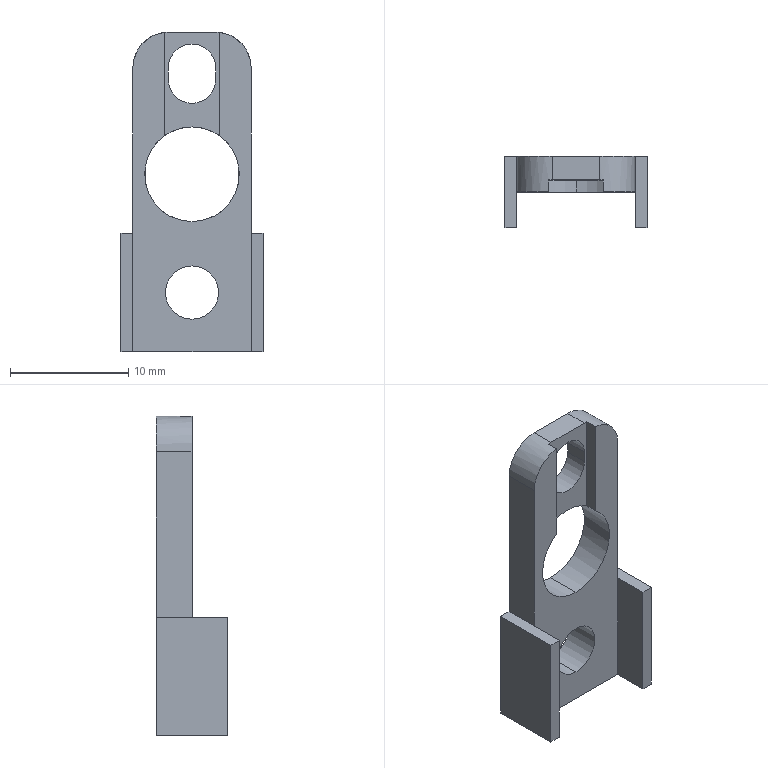Component | SolidWorks | BearingHousingAssembly-1_JawBuckleJaw-1 | 1 solid | 28 faces | box 12 x 6 x 27 mm | volume 649 mm3 | plane 19 | cylinder 9 | commonest cylinder face diameters 4 x3 8 x2 4.5 x2 6 x2
build123d program:
from build123d import *

# Parameters (mm, degrees)
SKETCH1_W                  = 27
SKETCH1_H                  = 10
BOSS_EXTRUDE1_DEPTH        = 3
F_4_5_4_5_DIAMETER_HOLE1_D = 4.5
SKETCH4_W                  = 6
SKETCH4_H                  = 1
BOSS_EXTRUDE2_DEPTH        = 10
SKETCH5_R                  = 4
CUT_EXTRUDE1_DEPTH         = 29.302
FILLET1_R                  = 3
CUT_EXTRUDE2_DEPTH         = 29.302
SKETCH7_W                  = 10.742
SKETCH7_H                  = 4.6
CUT_EXTRUDE3_DEPTH         = 1


with BuildPart() as part:
    # Sketch1 → Boss-Extrude1 (new body)
    with BuildSketch(Plane.XY):
        with Locations((13.5, 0)):
            Rectangle(SKETCH1_W, SKETCH1_H)
    extrude(amount=BOSS_EXTRUDE1_DEPTH)

    # 4.5 _4.5_ Diameter Hole1 (through all)
    with Locations(Plane(origin=(0, 0, 0), x_dir=(-1, 0, 0), z_dir=(0, 0, -1))):
        with Locations((-5, 0)):
            Hole(F_4_5_4_5_DIAMETER_HOLE1_D / 2)

    # Sketch4 → Boss-Extrude2 (add)
    with BuildSketch(Plane.ZY):
        with Locations((0, 5.5)):
            Rectangle(SKETCH4_W, SKETCH4_H)
        with Locations((0, -5.5)):
            Rectangle(SKETCH4_W, SKETCH4_H)
    extrude(amount=-BOSS_EXTRUDE2_DEPTH)

    # Sketch5 → Cut-Extrude1 (cut, through all)
    with BuildSketch(Plane.XY.offset(3)):
        with Locations((15, 0)):
            Circle(SKETCH5_R)
    extrude(amount=-CUT_EXTRUDE1_DEPTH, mode=Mode.SUBTRACT)

    # Fillet1
    fillet1_edges = [part.edges().sort_by_distance(p)[0] for p in [
        (27, -5, 1.5),
        (27, 5, 1.5),
    ]]
    fillet(fillet1_edges, radius=FILLET1_R)

    # Sketch6 → Cut-Extrude2 (cut, through all)
    with BuildSketch(Plane.XY.offset(3)):
        with BuildLine():
            Line((23, 2), (24, 2))
            ThreePointArc((24, 2), (26, 0), (24, -2))
            Line((24, -2), (23, -2))
            ThreePointArc((23, -2), (21, 0), (23, 2))
        make_face()
    extrude(amount=-CUT_EXTRUDE2_DEPTH, mode=Mode.SUBTRACT)

    # Sketch7 → Cut-Extrude3 (cut)
    with BuildSketch(Plane(origin=(0, 0, 0), x_dir=(-1, 0, 0), z_dir=(0, 0, -1))):
        with Locations((-23.371, 0)):
            Rectangle(SKETCH7_W, SKETCH7_H)
    extrude(amount=-CUT_EXTRUDE3_DEPTH, mode=Mode.SUBTRACT)


solid = part.part

# Placed as in the assembly
solid = solid.moved(Location((-38.666, 349.464, -16), (-90, 0, -90)))
STEP:
#1=COLOUR_RGB('',0.7922,0.8196,0.9333);
#2=FILL_AREA_STYLE_COLOUR('',#1);
#3=FILL_AREA_STYLE('',(#2));
#4=SURFACE_STYLE_FILL_AREA(#3);
#5=SURFACE_SIDE_STYLE('',(#4));
#6=SURFACE_STYLE_USAGE(.BOTH.,#5);
#7=PRESENTATION_STYLE_ASSIGNMENT((#6));
#8=CARTESIAN_POINT('',(-1.522,13.758,-0.1969));
#9=VERTEX_POINT('',#8);
#10=CARTESIAN_POINT('',(-1.613,13.758,0.08947));
#11=VERTEX_POINT('',#10);
#12=CARTESIAN_POINT('',(-1.522,13.758,-0.03937));
#13=DIRECTION('',(0.,1.,0.));
#14=DIRECTION('',(0.,0.,1.));
#15=AXIS2_PLACEMENT_3D('',#12,#13,#14);
#16=CIRCLE('',#15,0.1575);
#17=EDGE_CURVE('',#9,#11,#16,.T.);
#18=ORIENTED_EDGE('',*,*,#17,.F.);
#19=CARTESIAN_POINT('',(-1.522,13.877,-0.1969));
#20=VERTEX_POINT('',#19);
#21=CARTESIAN_POINT('',(-1.522,13.64,-0.1969));
#22=DIRECTION('',(0.,1.,0.));
#23=VECTOR('',#22,39.37);
#24=LINE('',#21,#23);
#25=EDGE_CURVE('',#9,#20,#24,.T.);
#26=ORIENTED_EDGE('',*,*,#25,.T.);
#27=CARTESIAN_POINT('',(-1.522,13.877,0.1181));
#28=VERTEX_POINT('',#27);
#29=CARTESIAN_POINT('',(-1.522,13.877,-0.03937));
#30=DIRECTION('',(0.,1.,0.));
#31=DIRECTION('',(0.,0.,1.));
#32=AXIS2_PLACEMENT_3D('',#29,#30,#31);
#33=CIRCLE('',#32,0.1575);
#34=EDGE_CURVE('',#20,#28,#33,.T.);
#35=ORIENTED_EDGE('',*,*,#34,.T.);
#36=CARTESIAN_POINT('',(-1.522,13.798,0.1181));
#37=VERTEX_POINT('',#36);
#38=CARTESIAN_POINT('',(-1.522,13.64,0.1181));
#39=DIRECTION('',(0.,1.,0.));
#40=VECTOR('',#39,39.37);
#41=LINE('',#38,#40);
#42=EDGE_CURVE('',#37,#28,#41,.T.);
#43=ORIENTED_EDGE('',*,*,#42,.F.);
#44=CARTESIAN_POINT('',(-1.613,13.798,0.08947));
#45=VERTEX_POINT('',#44);
#46=CARTESIAN_POINT('',(-1.522,13.798,-0.03937));
#47=DIRECTION('',(0.,1.,0.));
#48=DIRECTION('',(-0.,0.,-1.));
#49=AXIS2_PLACEMENT_3D('',#46,#47,#48);
#50=CIRCLE('',#49,0.1575);
#51=EDGE_CURVE('',#45,#37,#50,.T.);
#52=ORIENTED_EDGE('',*,*,#51,.F.);
#53=CARTESIAN_POINT('',(-1.613,13.64,0.08947));
#54=DIRECTION('',(-0.,-1.,-0.));
#55=VECTOR('',#54,39.37);
#56=LINE('',#53,#55);
#57=EDGE_CURVE('',#45,#11,#56,.T.);
#58=ORIENTED_EDGE('',*,*,#57,.T.);
#59=EDGE_LOOP('',(#18,#26,#35,#43,#52,#58));
#60=FACE_OUTER_BOUND('',#59,.T.);
#61=CARTESIAN_POINT('',(-1.522,13.64,-0.03937));
#62=DIRECTION('',(0.,1.,0.));
#63=DIRECTION('',(0.,0.,1.));
#64=AXIS2_PLACEMENT_3D('',#61,#62,#63);
#65=CYLINDRICAL_SURFACE('',#64,0.1575);
#66=ADVANCED_FACE('',(#60),#65,.F.);
#67=CARTESIAN_POINT('',(-1.522,13.877,-0.3445));
#68=VERTEX_POINT('',#67);
#69=CARTESIAN_POINT('',(-1.522,13.877,-0.5217));
#70=VERTEX_POINT('',#69);
#71=CARTESIAN_POINT('',(-1.522,13.877,-0.4331));
#72=DIRECTION('',(-0.,-1.,-0.));
#73=DIRECTION('',(-0.,0.,-1.));
#74=AXIS2_PLACEMENT_3D('',#71,#72,#73);
#75=CIRCLE('',#74,0.08858);
#76=EDGE_CURVE('',#68,#70,#75,.T.);
#77=ORIENTED_EDGE('',*,*,#76,.F.);
#78=CARTESIAN_POINT('',(-1.522,13.758,-0.3445));
#79=VERTEX_POINT('',#78);
#80=CARTESIAN_POINT('',(-1.522,13.758,-0.3445));
#81=DIRECTION('',(-0.,-1.,-0.));
#82=VECTOR('',#81,39.37);
#83=LINE('',#80,#82);
#84=EDGE_CURVE('',#68,#79,#83,.T.);
#85=ORIENTED_EDGE('',*,*,#84,.T.);
#86=CARTESIAN_POINT('',(-1.522,13.758,-0.5217));
#87=VERTEX_POINT('',#86);
#88=CARTESIAN_POINT('',(-1.522,13.758,-0.4331));
#89=DIRECTION('',(-0.,-1.,-0.));
#90=DIRECTION('',(-0.,0.,-1.));
#91=AXIS2_PLACEMENT_3D('',#88,#89,#90);
#92=CIRCLE('',#91,0.08858);
#93=EDGE_CURVE('',#79,#87,#92,.T.);
#94=ORIENTED_EDGE('',*,*,#93,.T.);
#95=CARTESIAN_POINT('',(-1.522,13.758,-0.5217));
#96=DIRECTION('',(-0.,-1.,-0.));
#97=VECTOR('',#96,39.37);
#98=LINE('',#95,#97);
#99=EDGE_CURVE('',#70,#87,#98,.T.);
#100=ORIENTED_EDGE('',*,*,#99,.F.);
#101=EDGE_LOOP('',(#77,#85,#94,#100));
#102=FACE_OUTER_BOUND('',#101,.T.);
#103=CARTESIAN_POINT('',(-1.522,13.758,-0.4331));
#104=DIRECTION('',(-0.,-1.,-0.));
#105=DIRECTION('',(-0.,0.,-1.));
#106=AXIS2_PLACEMENT_3D('',#103,#104,#105);
#107=CYLINDRICAL_SURFACE('',#106,0.08858);
#108=ADVANCED_FACE('',(#102),#107,.F.);
#109=CARTESIAN_POINT('',(-1.522,13.798,0.3937));
#110=VERTEX_POINT('',#109);
#111=CARTESIAN_POINT('',(-1.444,13.798,0.315));
#112=VERTEX_POINT('',#111);
#113=CARTESIAN_POINT('',(-1.522,13.798,0.315));
#114=DIRECTION('',(0.,1.,0.));
#115=DIRECTION('',(-0.,0.,-1.));
#116=AXIS2_PLACEMENT_3D('',#113,#114,#115);
#117=CIRCLE('',#116,0.07874);
#118=EDGE_CURVE('',#110,#112,#117,.T.);
#119=ORIENTED_EDGE('',*,*,#118,.F.);
#120=CARTESIAN_POINT('',(-1.522,13.877,0.3937));
#121=VERTEX_POINT('',#120);
#122=CARTESIAN_POINT('',(-1.522,13.64,0.3937));
#123=DIRECTION('',(0.,1.,0.));
#124=VECTOR('',#123,39.37);
#125=LINE('',#122,#124);
#126=EDGE_CURVE('',#110,#121,#125,.T.);
#127=ORIENTED_EDGE('',*,*,#126,.T.);
#128=CARTESIAN_POINT('',(-1.444,13.877,0.315));
#129=VERTEX_POINT('',#128);
#130=CARTESIAN_POINT('',(-1.522,13.877,0.315));
#131=DIRECTION('',(0.,1.,0.));
#132=DIRECTION('',(0.,0.,1.));
#133=AXIS2_PLACEMENT_3D('',#130,#131,#132);
#134=CIRCLE('',#133,0.07874);
#135=EDGE_CURVE('',#121,#129,#134,.T.);
#136=ORIENTED_EDGE('',*,*,#135,.T.);
#137=CARTESIAN_POINT('',(-1.444,13.64,0.315));
#138=DIRECTION('',(0.,1.,0.));
#139=VECTOR('',#138,39.37);
#140=LINE('',#137,#139);
#141=EDGE_CURVE('',#112,#129,#140,.T.);
#142=ORIENTED_EDGE('',*,*,#141,.F.);
#143=EDGE_LOOP('',(#119,#127,#136,#142));
#144=FACE_OUTER_BOUND('',#143,.T.);
#145=CARTESIAN_POINT('',(-1.522,13.64,0.315));
#146=DIRECTION('',(0.,1.,0.));
#147=DIRECTION('',(0.,0.,1.));
#148=AXIS2_PLACEMENT_3D('',#145,#146,#147);
#149=CYLINDRICAL_SURFACE('',#148,0.07874);
#150=ADVANCED_FACE('',(#144),#149,.F.);
#151=CARTESIAN_POINT('',(-1.444,13.798,0.4331));
#152=VERTEX_POINT('',#151);
#153=CARTESIAN_POINT('',(-1.601,13.798,0.4331));
#154=VERTEX_POINT('',#153);
#155=CARTESIAN_POINT('',(-1.325,13.798,0.4331));
#156=DIRECTION('',(-1.,0.,0.));
#157=VECTOR('',#156,39.37);
#158=LINE('',#155,#157);
#159=EDGE_CURVE('',#152,#154,#158,.T.);
#160=ORIENTED_EDGE('',*,*,#159,.F.);
#161=CARTESIAN_POINT('',(-1.444,13.877,0.4331));
#162=VERTEX_POINT('',#161);
#163=CARTESIAN_POINT('',(-1.444,13.877,0.4331));
#164=DIRECTION('',(0.,1.,0.));
#165=VECTOR('',#164,39.37);
#166=LINE('',#163,#165);
#167=EDGE_CURVE('',#152,#162,#166,.T.);
#168=ORIENTED_EDGE('',*,*,#167,.T.);
#169=CARTESIAN_POINT('',(-1.601,13.877,0.4331));
#170=VERTEX_POINT('',#169);
#171=CARTESIAN_POINT('',(-1.325,13.877,0.4331));
#172=DIRECTION('',(1.,-0.,-0.));
#173=VECTOR('',#172,39.37);
#174=LINE('',#171,#173);
#175=EDGE_CURVE('',#170,#162,#174,.T.);
#176=ORIENTED_EDGE('',*,*,#175,.F.);
#177=CARTESIAN_POINT('',(-1.601,13.877,0.4331));
#178=DIRECTION('',(-0.,-1.,-0.));
#179=VECTOR('',#178,39.37);
#180=LINE('',#177,#179);
#181=EDGE_CURVE('',#170,#154,#180,.T.);
#182=ORIENTED_EDGE('',*,*,#181,.T.);
#183=EDGE_LOOP('',(#160,#168,#176,#182));
#184=FACE_OUTER_BOUND('',#183,.T.);
#185=CARTESIAN_POINT('',(-1.325,13.877,0.4331));
#186=DIRECTION('',(-0.,0.,-1.));
#187=DIRECTION('',(0.,1.,0.));
#188=AXIS2_PLACEMENT_3D('',#185,#186,#187);
#189=PLANE('',#188);
#190=ADVANCED_FACE('',(#184),#189,.F.);
#191=CARTESIAN_POINT('',(-1.444,13.798,0.2756));
#192=VERTEX_POINT('',#191);
#193=CARTESIAN_POINT('',(-1.601,13.798,0.2756));
#194=VERTEX_POINT('',#193);
#195=CARTESIAN_POINT('',(-1.522,13.798,0.2756));
#196=DIRECTION('',(0.,1.,0.));
#197=DIRECTION('',(-0.,0.,-1.));
#198=AXIS2_PLACEMENT_3D('',#195,#196,#197);
#199=CIRCLE('',#198,0.07874);
#200=EDGE_CURVE('',#192,#194,#199,.T.);
#201=ORIENTED_EDGE('',*,*,#200,.F.);
#202=CARTESIAN_POINT('',(-1.444,13.877,0.2756));
#203=VERTEX_POINT('',#202);
#204=CARTESIAN_POINT('',(-1.444,13.64,0.2756));
#205=DIRECTION('',(0.,1.,0.));
#206=VECTOR('',#205,39.37);
#207=LINE('',#204,#206);
#208=EDGE_CURVE('',#192,#203,#207,.T.);
#209=ORIENTED_EDGE('',*,*,#208,.T.);
#210=CARTESIAN_POINT('',(-1.601,13.877,0.2756));
#211=VERTEX_POINT('',#210);
#212=CARTESIAN_POINT('',(-1.522,13.877,0.2756));
#213=DIRECTION('',(0.,1.,0.));
#214=DIRECTION('',(0.,0.,1.));
#215=AXIS2_PLACEMENT_3D('',#212,#213,#214);
#216=CIRCLE('',#215,0.07874);
#217=EDGE_CURVE('',#203,#211,#216,.T.);
#218=ORIENTED_EDGE('',*,*,#217,.T.);
#219=CARTESIAN_POINT('',(-1.601,13.64,0.2756));
#220=DIRECTION('',(0.,1.,0.));
#221=VECTOR('',#220,39.37);
#222=LINE('',#219,#221);
#223=EDGE_CURVE('',#194,#211,#222,.T.);
#224=ORIENTED_EDGE('',*,*,#223,.F.);
#225=EDGE_LOOP('',(#201,#209,#218,#224));
#226=FACE_OUTER_BOUND('',#225,.T.);
#227=CARTESIAN_POINT('',(-1.522,13.64,0.2756));
#228=DIRECTION('',(0.,1.,0.));
#229=DIRECTION('',(0.,0.,1.));
#230=AXIS2_PLACEMENT_3D('',#227,#228,#229);
#231=CYLINDRICAL_SURFACE('',#230,0.07874);
#232=ADVANCED_FACE('',(#226),#231,.F.);
#233=CARTESIAN_POINT('',(-1.444,13.798,0.2756));
#234=DIRECTION('',(-0.,0.,-1.));
#235=VECTOR('',#234,39.37);
#236=LINE('',#233,#235);
#237=EDGE_CURVE('',#112,#192,#236,.T.);
#238=ORIENTED_EDGE('',*,*,#237,.F.);
#239=ORIENTED_EDGE('',*,*,#141,.T.);
#240=CARTESIAN_POINT('',(-1.444,13.877,0.2756));
#241=DIRECTION('',(-0.,0.,-1.));
#242=VECTOR('',#241,39.37);
#243=LINE('',#240,#242);
#244=EDGE_CURVE('',#129,#203,#243,.T.);
#245=ORIENTED_EDGE('',*,*,#244,.T.);
#246=ORIENTED_EDGE('',*,*,#208,.F.);
#247=EDGE_LOOP('',(#238,#239,#245,#246));
#248=FACE_OUTER_BOUND('',#247,.T.);
#249=CARTESIAN_POINT('',(-1.444,13.64,0.2756));
#250=DIRECTION('',(1.,-0.,-0.));
#251=DIRECTION('',(0.,1.,0.));
#252=AXIS2_PLACEMENT_3D('',#249,#250,#251);
#253=PLANE('',#252);
#254=ADVANCED_FACE('',(#248),#253,.F.);
#255=ORIENTED_EDGE('',*,*,#126,.F.);
#256=CARTESIAN_POINT('',(-1.601,13.798,0.315));
#257=VERTEX_POINT('',#256);
#258=CARTESIAN_POINT('',(-1.522,13.798,0.315));
#259=DIRECTION('',(0.,1.,0.));
#260=DIRECTION('',(-0.,0.,-1.));
#261=AXIS2_PLACEMENT_3D('',#258,#259,#260);
#262=CIRCLE('',#261,0.07874);
#263=EDGE_CURVE('',#257,#110,#262,.T.);
#264=ORIENTED_EDGE('',*,*,#263,.F.);
#265=CARTESIAN_POINT('',(-1.601,13.877,0.315));
#266=VERTEX_POINT('',#265);
#267=CARTESIAN_POINT('',(-1.601,13.64,0.315));
#268=DIRECTION('',(0.,1.,0.));
#269=VECTOR('',#268,39.37);
#270=LINE('',#267,#269);
#271=EDGE_CURVE('',#257,#266,#270,.T.);
#272=ORIENTED_EDGE('',*,*,#271,.T.);
#273=CARTESIAN_POINT('',(-1.522,13.877,0.315));
#274=DIRECTION('',(0.,1.,0.));
#275=DIRECTION('',(0.,0.,1.));
#276=AXIS2_PLACEMENT_3D('',#273,#274,#275);
#277=CIRCLE('',#276,0.07874);
#278=EDGE_CURVE('',#266,#121,#277,.T.);
#279=ORIENTED_EDGE('',*,*,#278,.T.);
#280=EDGE_LOOP('',(#255,#264,#272,#279));
#281=FACE_OUTER_BOUND('',#280,.T.);
#282=CARTESIAN_POINT('',(-1.522,13.64,0.315));
#283=DIRECTION('',(0.,1.,0.));
#284=DIRECTION('',(0.,0.,1.));
#285=AXIS2_PLACEMENT_3D('',#282,#283,#284);
#286=CYLINDRICAL_SURFACE('',#285,0.07874);
#287=ADVANCED_FACE('',(#281),#286,.F.);
#288=CARTESIAN_POINT('',(-1.601,13.798,0.2756));
#289=DIRECTION('',(0.,-0.,1.));
#290=VECTOR('',#289,39.37);
#291=LINE('',#288,#290);
#292=EDGE_CURVE('',#194,#257,#291,.T.);
#293=ORIENTED_EDGE('',*,*,#292,.F.);
#294=ORIENTED_EDGE('',*,*,#223,.T.);
#295=CARTESIAN_POINT('',(-1.601,13.877,0.2756));
#296=DIRECTION('',(0.,-0.,1.));
#297=VECTOR('',#296,39.37);
#298=LINE('',#295,#297);
#299=EDGE_CURVE('',#211,#266,#298,.T.);
#300=ORIENTED_EDGE('',*,*,#299,.T.);
#301=ORIENTED_EDGE('',*,*,#271,.F.);
#302=EDGE_LOOP('',(#293,#294,#300,#301));
#303=FACE_OUTER_BOUND('',#302,.T.);
#304=CARTESIAN_POINT('',(-1.601,13.64,0.2756));
#305=DIRECTION('',(-1.,0.,0.));
#306=DIRECTION('',(-0.,-1.,-0.));
#307=AXIS2_PLACEMENT_3D('',#304,#305,#306);
#308=PLANE('',#307);
#309=ADVANCED_FACE('',(#303),#308,.F.);
#310=CARTESIAN_POINT('',(-1.325,13.758,-0.6299));
#311=VERTEX_POINT('',#310);
#312=CARTESIAN_POINT('',(-1.719,13.758,-0.6299));
#313=VERTEX_POINT('',#312);
#314=CARTESIAN_POINT('',(-1.325,13.758,-0.6299));
#315=DIRECTION('',(-1.,0.,0.));
#316=VECTOR('',#315,39.37);
#317=LINE('',#314,#316);
#318=EDGE_CURVE('',#311,#313,#317,.T.);
#319=ORIENTED_EDGE('',*,*,#318,.T.);
#320=CARTESIAN_POINT('',(-1.719,13.64,-0.6299));
#321=VERTEX_POINT('',#320);
#322=CARTESIAN_POINT('',(-1.719,13.877,-0.6299));
#323=DIRECTION('',(-0.,-1.,-0.));
#324=VECTOR('',#323,39.37);
#325=LINE('',#322,#324);
#326=EDGE_CURVE('',#313,#321,#325,.T.);
#327=ORIENTED_EDGE('',*,*,#326,.T.);
#328=CARTESIAN_POINT('',(-1.758,13.64,-0.6299));
#329=VERTEX_POINT('',#328);
#330=CARTESIAN_POINT('',(-1.719,13.64,-0.6299));
#331=DIRECTION('',(-1.,0.,0.));
#332=VECTOR('',#331,39.37);
#333=LINE('',#330,#332);
#334=EDGE_CURVE('',#321,#329,#333,.T.);
#335=ORIENTED_EDGE('',*,*,#334,.T.);
#336=CARTESIAN_POINT('',(-1.758,13.877,-0.6299));
#337=VERTEX_POINT('',#336);
#338=CARTESIAN_POINT('',(-1.758,13.877,-0.6299));
#339=DIRECTION('',(0.,1.,0.));
#340=VECTOR('',#339,39.37);
#341=LINE('',#338,#340);
#342=EDGE_CURVE('',#329,#337,#341,.T.);
#343=ORIENTED_EDGE('',*,*,#342,.T.);
#344=CARTESIAN_POINT('',(-1.286,13.877,-0.6299));
#345=VERTEX_POINT('',#344);
#346=CARTESIAN_POINT('',(-1.325,13.877,-0.6299));
#347=DIRECTION('',(-1.,0.,0.));
#348=VECTOR('',#347,39.37);
#349=LINE('',#346,#348);
#350=EDGE_CURVE('',#345,#337,#349,.T.);
#351=ORIENTED_EDGE('',*,*,#350,.F.);
#352=CARTESIAN_POINT('',(-1.286,13.64,-0.6299));
#353=VERTEX_POINT('',#352);
#354=CARTESIAN_POINT('',(-1.286,13.877,-0.6299));
#355=DIRECTION('',(-0.,-1.,-0.));
#356=VECTOR('',#355,39.37);
#357=LINE('',#354,#356);
#358=EDGE_CURVE('',#345,#353,#357,.T.);
#359=ORIENTED_EDGE('',*,*,#358,.T.);
#360=CARTESIAN_POINT('',(-1.325,13.64,-0.6299));
#361=VERTEX_POINT('',#360);
#362=CARTESIAN_POINT('',(-1.325,13.64,-0.6299));
#363=DIRECTION('',(-1.,0.,0.));
#364=VECTOR('',#363,39.37);
#365=LINE('',#362,#364);
#366=EDGE_CURVE('',#353,#361,#365,.T.);
#367=ORIENTED_EDGE('',*,*,#366,.T.);
#368=CARTESIAN_POINT('',(-1.325,13.877,-0.6299));
#369=DIRECTION('',(0.,1.,0.));
#370=VECTOR('',#369,39.37);
#371=LINE('',#368,#370);
#372=EDGE_CURVE('',#361,#311,#371,.T.);
#373=ORIENTED_EDGE('',*,*,#372,.T.);
#374=EDGE_LOOP('',(#319,#327,#335,#343,#351,#359,#367,#373));
#375=FACE_OUTER_BOUND('',#374,.T.);
#376=CARTESIAN_POINT('',(-1.325,13.877,-0.6299));
#377=DIRECTION('',(0.,-0.,1.));
#378=DIRECTION('',(1.,-0.,-0.));
#379=AXIS2_PLACEMENT_3D('',#376,#377,#378);
#380=PLANE('',#379);
#381=ADVANCED_FACE('',(#375),#380,.F.);
#382=CARTESIAN_POINT('',(-1.719,13.758,-0.2362));
#383=VERTEX_POINT('',#382);
#384=CARTESIAN_POINT('',(-1.719,13.758,0.315));
#385=VERTEX_POINT('',#384);
#386=CARTESIAN_POINT('',(-1.719,13.758,-0.6299));
#387=DIRECTION('',(0.,-0.,1.));
#388=VECTOR('',#387,39.37);
#389=LINE('',#386,#388);
#390=EDGE_CURVE('',#383,#385,#389,.T.);
#391=ORIENTED_EDGE('',*,*,#390,.T.);
#392=CARTESIAN_POINT('',(-1.719,13.877,0.315));
#393=VERTEX_POINT('',#392);
#394=CARTESIAN_POINT('',(-1.719,13.877,0.315));
#395=DIRECTION('',(0.,1.,0.));
#396=VECTOR('',#395,39.37);
#397=LINE('',#394,#396);
#398=EDGE_CURVE('',#385,#393,#397,.T.);
#399=ORIENTED_EDGE('',*,*,#398,.T.);
#400=CARTESIAN_POINT('',(-1.719,13.877,-0.2362));
#401=VERTEX_POINT('',#400);
#402=CARTESIAN_POINT('',(-1.719,13.877,-0.6299));
#403=DIRECTION('',(0.,-0.,1.));
#404=VECTOR('',#403,39.37);
#405=LINE('',#402,#404);
#406=EDGE_CURVE('',#401,#393,#405,.T.);
#407=ORIENTED_EDGE('',*,*,#406,.F.);
#408=CARTESIAN_POINT('',(-1.719,13.877,-0.2362));
#409=DIRECTION('',(-0.,-1.,-0.));
#410=VECTOR('',#409,39.37);
#411=LINE('',#408,#410);
#412=EDGE_CURVE('',#401,#383,#411,.T.);
#413=ORIENTED_EDGE('',*,*,#412,.T.);
#414=EDGE_LOOP('',(#391,#399,#407,#413));
#415=FACE_OUTER_BOUND('',#414,.T.);
#416=CARTESIAN_POINT('',(-1.719,13.877,-0.6299));
#417=DIRECTION('',(1.,-0.,-0.));
#418=DIRECTION('',(0.,1.,0.));
#419=AXIS2_PLACEMENT_3D('',#416,#417,#418);
#420=PLANE('',#419);
#421=ADVANCED_FACE('',(#415),#420,.F.);
#422=CARTESIAN_POINT('',(-1.325,13.877,0.315));
#423=VERTEX_POINT('',#422);
#424=CARTESIAN_POINT('',(-1.325,13.877,-0.2362));
#425=VERTEX_POINT('',#424);
#426=CARTESIAN_POINT('',(-1.325,13.877,-0.6299));
#427=DIRECTION('',(-0.,0.,-1.));
#428=VECTOR('',#427,39.37);
#429=LINE('',#426,#428);
#430=EDGE_CURVE('',#423,#425,#429,.T.);
#431=ORIENTED_EDGE('',*,*,#430,.F.);
#432=CARTESIAN_POINT('',(-1.325,13.758,0.315));
#433=VERTEX_POINT('',#432);
#434=CARTESIAN_POINT('',(-1.325,13.877,0.315));
#435=DIRECTION('',(-0.,-1.,-0.));
#436=VECTOR('',#435,39.37);
#437=LINE('',#434,#436);
#438=EDGE_CURVE('',#423,#433,#437,.T.);
#439=ORIENTED_EDGE('',*,*,#438,.T.);
#440=CARTESIAN_POINT('',(-1.325,13.758,-0.2362));
#441=VERTEX_POINT('',#440);
#442=CARTESIAN_POINT('',(-1.325,13.758,-0.6299));
#443=DIRECTION('',(-0.,0.,-1.));
#444=VECTOR('',#443,39.37);
#445=LINE('',#442,#444);
#446=EDGE_CURVE('',#433,#441,#445,.T.);
#447=ORIENTED_EDGE('',*,*,#446,.T.);
#448=CARTESIAN_POINT('',(-1.325,13.877,-0.2362));
#449=DIRECTION('',(0.,1.,0.));
#450=VECTOR('',#449,39.37);
#451=LINE('',#448,#450);
#452=EDGE_CURVE('',#441,#425,#451,.T.);
#453=ORIENTED_EDGE('',*,*,#452,.T.);
#454=EDGE_LOOP('',(#431,#439,#447,#453));
#455=FACE_OUTER_BOUND('',#454,.T.);
#456=CARTESIAN_POINT('',(-1.325,13.877,-0.6299));
#457=DIRECTION('',(-1.,0.,0.));
#458=DIRECTION('',(-0.,-1.,-0.));
#459=AXIS2_PLACEMENT_3D('',#456,#457,#458);
#460=PLANE('',#459);
#461=ADVANCED_FACE('',(#455),#460,.F.);
#462=ORIENTED_EDGE('',*,*,#217,.F.);
#463=ORIENTED_EDGE('',*,*,#244,.F.);
#464=ORIENTED_EDGE('',*,*,#135,.F.);
#465=ORIENTED_EDGE('',*,*,#278,.F.);
#466=ORIENTED_EDGE('',*,*,#299,.F.);
#467=EDGE_LOOP('',(#462,#463,#464,#465,#466));
#468=FACE_BOUND('',#467,.T.);
#469=CARTESIAN_POINT('',(-1.522,13.877,-0.03937));
#470=DIRECTION('',(0.,1.,0.));
#471=DIRECTION('',(0.,0.,1.));
#472=AXIS2_PLACEMENT_3D('',#469,#470,#471);
#473=CIRCLE('',#472,0.1575);
#474=EDGE_CURVE('',#28,#20,#473,.T.);
#475=ORIENTED_EDGE('',*,*,#474,.F.);
#476=ORIENTED_EDGE('',*,*,#34,.F.);
#477=EDGE_LOOP('',(#475,#476));
#478=FACE_BOUND('',#477,.T.);
#479=CARTESIAN_POINT('',(-1.522,13.877,-0.4331));
#480=DIRECTION('',(-0.,-1.,-0.));
#481=DIRECTION('',(-0.,0.,-1.));
#482=AXIS2_PLACEMENT_3D('',#479,#480,#481);
#483=CIRCLE('',#482,0.08858);
#484=EDGE_CURVE('',#70,#68,#483,.T.);
#485=ORIENTED_EDGE('',*,*,#484,.T.);
#486=ORIENTED_EDGE('',*,*,#76,.T.);
#487=EDGE_LOOP('',(#485,#486));
#488=FACE_BOUND('',#487,.T.);
#489=ORIENTED_EDGE('',*,*,#406,.T.);
#490=CARTESIAN_POINT('',(-1.601,13.877,0.315));
#491=DIRECTION('',(0.,1.,0.));
#492=DIRECTION('',(0.,0.,1.));
#493=AXIS2_PLACEMENT_3D('',#490,#491,#492);
#494=CIRCLE('',#493,0.1181);
#495=EDGE_CURVE('',#393,#170,#494,.T.);
#496=ORIENTED_EDGE('',*,*,#495,.T.);
#497=ORIENTED_EDGE('',*,*,#175,.T.);
#498=CARTESIAN_POINT('',(-1.444,13.877,0.315));
#499=DIRECTION('',(0.,1.,0.));
#500=DIRECTION('',(0.,0.,1.));
#501=AXIS2_PLACEMENT_3D('',#498,#499,#500);
#502=CIRCLE('',#501,0.1181);
#503=EDGE_CURVE('',#162,#423,#502,.T.);
#504=ORIENTED_EDGE('',*,*,#503,.T.);
#505=ORIENTED_EDGE('',*,*,#430,.T.);
#506=CARTESIAN_POINT('',(-1.286,13.877,-0.2362));
#507=VERTEX_POINT('',#506);
#508=CARTESIAN_POINT('',(-1.325,13.877,-0.2362));
#509=DIRECTION('',(1.,-0.,-0.));
#510=VECTOR('',#509,39.37);
#511=LINE('',#508,#510);
#512=EDGE_CURVE('',#425,#507,#511,.T.);
#513=ORIENTED_EDGE('',*,*,#512,.T.);
#514=CARTESIAN_POINT('',(-1.286,13.877,-0.2362));
#515=DIRECTION('',(-0.,0.,-1.));
#516=VECTOR('',#515,39.37);
#517=LINE('',#514,#516);
#518=EDGE_CURVE('',#507,#345,#517,.T.);
#519=ORIENTED_EDGE('',*,*,#518,.T.);
#520=ORIENTED_EDGE('',*,*,#350,.T.);
#521=CARTESIAN_POINT('',(-1.758,13.877,-0.2362));
#522=VERTEX_POINT('',#521);
#523=CARTESIAN_POINT('',(-1.758,13.877,-0.2362));
#524=DIRECTION('',(-0.,0.,-1.));
#525=VECTOR('',#524,39.37);
#526=LINE('',#523,#525);
#527=EDGE_CURVE('',#522,#337,#526,.T.);
#528=ORIENTED_EDGE('',*,*,#527,.F.);
#529=CARTESIAN_POINT('',(-1.719,13.877,-0.2362));
#530=DIRECTION('',(1.,0.,-0.));
#531=VECTOR('',#530,39.37);
#532=LINE('',#529,#531);
#533=EDGE_CURVE('',#522,#401,#532,.T.);
#534=ORIENTED_EDGE('',*,*,#533,.T.);
#535=EDGE_LOOP('',(#489,#496,#497,#504,#505,#513,#519,#520,#528,#534));
#536=FACE_OUTER_BOUND('',#535,.T.);
#537=CARTESIAN_POINT('',(-1.522,13.877,-0.6299));
#538=DIRECTION('',(0.,1.,0.));
#539=DIRECTION('',(0.,-0.,1.));
#540=AXIS2_PLACEMENT_3D('',#537,#538,#539);
#541=PLANE('',#540);
#542=ADVANCED_FACE('',(#468,#478,#488,#536),#541,.T.);
#543=CARTESIAN_POINT('',(-1.432,13.758,0.4325));
#544=VERTEX_POINT('',#543);
#545=CARTESIAN_POINT('',(-1.444,13.758,0.315));
#546=DIRECTION('',(-0.,-1.,-0.));
#547=DIRECTION('',(0.,0.,1.));
#548=AXIS2_PLACEMENT_3D('',#545,#546,#547);
#549=CIRCLE('',#548,0.1181);
#550=EDGE_CURVE('',#433,#544,#549,.T.);
#551=ORIENTED_EDGE('',*,*,#550,.T.);
#552=CARTESIAN_POINT('',(-1.432,13.758,0.08947));
#553=VERTEX_POINT('',#552);
#554=CARTESIAN_POINT('',(-1.432,13.758,0.5016));
#555=DIRECTION('',(0.,-0.,1.));
#556=VECTOR('',#555,39.37);
#557=LINE('',#554,#556);
#558=EDGE_CURVE('',#553,#544,#557,.T.);
#559=ORIENTED_EDGE('',*,*,#558,.F.);
#560=CARTESIAN_POINT('',(-1.522,13.758,-0.03937));
#561=DIRECTION('',(0.,1.,0.));
#562=DIRECTION('',(0.,0.,1.));
#563=AXIS2_PLACEMENT_3D('',#560,#561,#562);
#564=CIRCLE('',#563,0.1575);
#565=EDGE_CURVE('',#553,#9,#564,.T.);
#566=ORIENTED_EDGE('',*,*,#565,.T.);
#567=ORIENTED_EDGE('',*,*,#17,.T.);
#568=CARTESIAN_POINT('',(-1.613,13.758,0.4325));
#569=VERTEX_POINT('',#568);
#570=CARTESIAN_POINT('',(-1.613,13.758,0.5016));
#571=DIRECTION('',(-0.,0.,-1.));
#572=VECTOR('',#571,39.37);
#573=LINE('',#570,#572);
#574=EDGE_CURVE('',#569,#11,#573,.T.);
#575=ORIENTED_EDGE('',*,*,#574,.F.);
#576=CARTESIAN_POINT('',(-1.601,13.758,0.315));
#577=DIRECTION('',(-0.,-1.,-0.));
#578=DIRECTION('',(0.,0.,1.));
#579=AXIS2_PLACEMENT_3D('',#576,#577,#578);
#580=CIRCLE('',#579,0.1181);
#581=EDGE_CURVE('',#569,#385,#580,.T.);
#582=ORIENTED_EDGE('',*,*,#581,.T.);
#583=ORIENTED_EDGE('',*,*,#390,.F.);
#584=CARTESIAN_POINT('',(-1.719,13.758,-0.6299));
#585=DIRECTION('',(0.,-0.,1.));
#586=VECTOR('',#585,39.37);
#587=LINE('',#584,#586);
#588=EDGE_CURVE('',#313,#383,#587,.T.);
#589=ORIENTED_EDGE('',*,*,#588,.F.);
#590=ORIENTED_EDGE('',*,*,#318,.F.);
#591=CARTESIAN_POINT('',(-1.325,13.758,-0.6299));
#592=DIRECTION('',(-0.,0.,-1.));
#593=VECTOR('',#592,39.37);
#594=LINE('',#591,#593);
#595=EDGE_CURVE('',#441,#311,#594,.T.);
#596=ORIENTED_EDGE('',*,*,#595,.F.);
#597=ORIENTED_EDGE('',*,*,#446,.F.);
#598=EDGE_LOOP('',(#551,#559,#566,#567,#575,#582,#583,#589,#590,#596,#597));
#599=FACE_OUTER_BOUND('',#598,.T.);
#600=CARTESIAN_POINT('',(-1.522,13.758,-0.4331));
#601=DIRECTION('',(-0.,-1.,-0.));
#602=DIRECTION('',(-0.,0.,-1.));
#603=AXIS2_PLACEMENT_3D('',#600,#601,#602);
#604=CIRCLE('',#603,0.08858);
#605=EDGE_CURVE('',#87,#79,#604,.T.);
#606=ORIENTED_EDGE('',*,*,#605,.F.);
#607=ORIENTED_EDGE('',*,*,#93,.F.);
#608=EDGE_LOOP('',(#606,#607));
#609=FACE_BOUND('',#608,.T.);
#610=CARTESIAN_POINT('',(-1.522,13.758,-0.6299));
#611=DIRECTION('',(0.,1.,0.));
#612=DIRECTION('',(0.,-0.,1.));
#613=AXIS2_PLACEMENT_3D('',#610,#611,#612);
#614=PLANE('',#613);
#615=ADVANCED_FACE('',(#599,#609),#614,.F.);
#616=ORIENTED_EDGE('',*,*,#84,.F.);
#617=ORIENTED_EDGE('',*,*,#484,.F.);
#618=ORIENTED_EDGE('',*,*,#99,.T.);
#619=ORIENTED_EDGE('',*,*,#605,.T.);
#620=EDGE_LOOP('',(#616,#617,#618,#619));
#621=FACE_OUTER_BOUND('',#620,.T.);
#622=CARTESIAN_POINT('',(-1.522,13.758,-0.4331));
#623=DIRECTION('',(-0.,-1.,-0.));
#624=DIRECTION('',(-0.,0.,-1.));
#625=AXIS2_PLACEMENT_3D('',#622,#623,#624);
#626=CYLINDRICAL_SURFACE('',#625,0.08858);
#627=ADVANCED_FACE('',(#621),#626,.F.);
#628=CARTESIAN_POINT('',(-1.325,13.64,-0.2362));
#629=VERTEX_POINT('',#628);
#630=CARTESIAN_POINT('',(-1.325,13.877,-0.2362));
#631=DIRECTION('',(0.,1.,0.));
#632=VECTOR('',#631,39.37);
#633=LINE('',#630,#632);
#634=EDGE_CURVE('',#629,#441,#633,.T.);
#635=ORIENTED_EDGE('',*,*,#634,.T.);
#636=ORIENTED_EDGE('',*,*,#595,.T.);
#637=ORIENTED_EDGE('',*,*,#372,.F.);
#638=CARTESIAN_POINT('',(-1.325,13.64,-0.2362));
#639=DIRECTION('',(-0.,0.,-1.));
#640=VECTOR('',#639,39.37);
#641=LINE('',#638,#640);
#642=EDGE_CURVE('',#629,#361,#641,.T.);
#643=ORIENTED_EDGE('',*,*,#642,.F.);
#644=EDGE_LOOP('',(#635,#636,#637,#643));
#645=FACE_OUTER_BOUND('',#644,.T.);
#646=CARTESIAN_POINT('',(-1.325,13.877,-0.2362));
#647=DIRECTION('',(-1.,0.,0.));
#648=DIRECTION('',(-0.,-1.,-0.));
#649=AXIS2_PLACEMENT_3D('',#646,#647,#648);
#650=PLANE('',#649);
#651=ADVANCED_FACE('',(#645),#650,.T.);
#652=ORIENTED_EDGE('',*,*,#366,.F.);
#653=CARTESIAN_POINT('',(-1.286,13.64,-0.2362));
#654=VERTEX_POINT('',#653);
#655=CARTESIAN_POINT('',(-1.286,13.64,-0.2362));
#656=DIRECTION('',(-0.,0.,-1.));
#657=VECTOR('',#656,39.37);
#658=LINE('',#655,#657);
#659=EDGE_CURVE('',#654,#353,#658,.T.);
#660=ORIENTED_EDGE('',*,*,#659,.F.);
#661=CARTESIAN_POINT('',(-1.325,13.64,-0.2362));
#662=DIRECTION('',(-1.,0.,0.));
#663=VECTOR('',#662,39.37);
#664=LINE('',#661,#663);
#665=EDGE_CURVE('',#654,#629,#664,.T.);
#666=ORIENTED_EDGE('',*,*,#665,.T.);
#667=ORIENTED_EDGE('',*,*,#642,.T.);
#668=EDGE_LOOP('',(#652,#660,#666,#667));
#669=FACE_OUTER_BOUND('',#668,.T.);
#670=CARTESIAN_POINT('',(-1.325,13.64,-0.2362));
#671=DIRECTION('',(-0.,-1.,-0.));
#672=DIRECTION('',(-0.,0.,-1.));
#673=AXIS2_PLACEMENT_3D('',#670,#671,#672);
#674=PLANE('',#673);
#675=ADVANCED_FACE('',(#669),#674,.T.);
#676=ORIENTED_EDGE('',*,*,#358,.F.);
#677=ORIENTED_EDGE('',*,*,#518,.F.);
#678=CARTESIAN_POINT('',(-1.286,13.877,-0.2362));
#679=DIRECTION('',(-0.,-1.,-0.));
#680=VECTOR('',#679,39.37);
#681=LINE('',#678,#680);
#682=EDGE_CURVE('',#507,#654,#681,.T.);
#683=ORIENTED_EDGE('',*,*,#682,.T.);
#684=ORIENTED_EDGE('',*,*,#659,.T.);
#685=EDGE_LOOP('',(#676,#677,#683,#684));
#686=FACE_OUTER_BOUND('',#685,.T.);
#687=CARTESIAN_POINT('',(-1.286,13.877,-0.2362));
#688=DIRECTION('',(1.,-0.,-0.));
#689=DIRECTION('',(0.,1.,0.));
#690=AXIS2_PLACEMENT_3D('',#687,#688,#689);
#691=PLANE('',#690);
#692=ADVANCED_FACE('',(#686),#691,.T.);
#693=ORIENTED_EDGE('',*,*,#512,.F.);
#694=ORIENTED_EDGE('',*,*,#452,.F.);
#695=ORIENTED_EDGE('',*,*,#634,.F.);
#696=ORIENTED_EDGE('',*,*,#665,.F.);
#697=ORIENTED_EDGE('',*,*,#682,.F.);
#698=EDGE_LOOP('',(#693,#694,#695,#696,#697));
#699=FACE_OUTER_BOUND('',#698,.T.);
#700=CARTESIAN_POINT('',(-1.522,13.758,-0.2362));
#701=DIRECTION('',(-0.,0.,-1.));
#702=DIRECTION('',(-1.,0.,0.));
#703=AXIS2_PLACEMENT_3D('',#700,#701,#702);
#704=PLANE('',#703);
#705=ADVANCED_FACE('',(#699),#704,.F.);
#706=ORIENTED_EDGE('',*,*,#342,.F.);
#707=CARTESIAN_POINT('',(-1.758,13.64,-0.2362));
#708=VERTEX_POINT('',#707);
#709=CARTESIAN_POINT('',(-1.758,13.64,-0.2362));
#710=DIRECTION('',(-0.,0.,-1.));
#711=VECTOR('',#710,39.37);
#712=LINE('',#709,#711);
#713=EDGE_CURVE('',#708,#329,#712,.T.);
#714=ORIENTED_EDGE('',*,*,#713,.F.);
#715=CARTESIAN_POINT('',(-1.758,13.877,-0.2362));
#716=DIRECTION('',(0.,1.,0.));
#717=VECTOR('',#716,39.37);
#718=LINE('',#715,#717);
#719=EDGE_CURVE('',#708,#522,#718,.T.);
#720=ORIENTED_EDGE('',*,*,#719,.T.);
#721=ORIENTED_EDGE('',*,*,#527,.T.);
#722=EDGE_LOOP('',(#706,#714,#720,#721));
#723=FACE_OUTER_BOUND('',#722,.T.);
#724=CARTESIAN_POINT('',(-1.758,13.877,-0.2362));
#725=DIRECTION('',(-1.,0.,0.));
#726=DIRECTION('',(-0.,-1.,-0.));
#727=AXIS2_PLACEMENT_3D('',#724,#725,#726);
#728=PLANE('',#727);
#729=ADVANCED_FACE('',(#723),#728,.T.);
#730=ORIENTED_EDGE('',*,*,#334,.F.);
#731=CARTESIAN_POINT('',(-1.719,13.64,-0.2362));
#732=VERTEX_POINT('',#731);
#733=CARTESIAN_POINT('',(-1.719,13.64,-0.2362));
#734=DIRECTION('',(-0.,0.,-1.));
#735=VECTOR('',#734,39.37);
#736=LINE('',#733,#735);
#737=EDGE_CURVE('',#732,#321,#736,.T.);
#738=ORIENTED_EDGE('',*,*,#737,.F.);
#739=CARTESIAN_POINT('',(-1.719,13.64,-0.2362));
#740=DIRECTION('',(-1.,0.,0.));
#741=VECTOR('',#740,39.37);
#742=LINE('',#739,#741);
#743=EDGE_CURVE('',#732,#708,#742,.T.);
#744=ORIENTED_EDGE('',*,*,#743,.T.);
#745=ORIENTED_EDGE('',*,*,#713,.T.);
#746=EDGE_LOOP('',(#730,#738,#744,#745));
#747=FACE_OUTER_BOUND('',#746,.T.);
#748=CARTESIAN_POINT('',(-1.719,13.64,-0.2362));
#749=DIRECTION('',(-0.,-1.,-0.));
#750=DIRECTION('',(1.,-0.,-0.));
#751=AXIS2_PLACEMENT_3D('',#748,#749,#750);
#752=PLANE('',#751);
#753=ADVANCED_FACE('',(#747),#752,.T.);
#754=ORIENTED_EDGE('',*,*,#326,.F.);
#755=ORIENTED_EDGE('',*,*,#588,.T.);
#756=CARTESIAN_POINT('',(-1.719,13.877,-0.2362));
#757=DIRECTION('',(-0.,-1.,-0.));
#758=VECTOR('',#757,39.37);
#759=LINE('',#756,#758);
#760=EDGE_CURVE('',#383,#732,#759,.T.);
#761=ORIENTED_EDGE('',*,*,#760,.T.);
#762=ORIENTED_EDGE('',*,*,#737,.T.);
#763=EDGE_LOOP('',(#754,#755,#761,#762));
#764=FACE_OUTER_BOUND('',#763,.T.);
#765=CARTESIAN_POINT('',(-1.719,13.877,-0.2362));
#766=DIRECTION('',(1.,-0.,-0.));
#767=DIRECTION('',(0.,1.,0.));
#768=AXIS2_PLACEMENT_3D('',#765,#766,#767);
#769=PLANE('',#768);
#770=ADVANCED_FACE('',(#764),#769,.T.);
#771=ORIENTED_EDGE('',*,*,#533,.F.);
#772=ORIENTED_EDGE('',*,*,#719,.F.);
#773=ORIENTED_EDGE('',*,*,#743,.F.);
#774=ORIENTED_EDGE('',*,*,#760,.F.);
#775=ORIENTED_EDGE('',*,*,#412,.F.);
#776=EDGE_LOOP('',(#771,#772,#773,#774,#775));
#777=FACE_OUTER_BOUND('',#776,.T.);
#778=CARTESIAN_POINT('',(-1.522,13.758,-0.2362));
#779=DIRECTION('',(0.,-0.,1.));
#780=DIRECTION('',(1.,-0.,-0.));
#781=AXIS2_PLACEMENT_3D('',#778,#779,#780);
#782=PLANE('',#781);
#783=ADVANCED_FACE('',(#777),#782,.T.);
#784=ORIENTED_EDGE('',*,*,#25,.F.);
#785=ORIENTED_EDGE('',*,*,#565,.F.);
#786=CARTESIAN_POINT('',(-1.432,13.798,0.08947));
#787=VERTEX_POINT('',#786);
#788=CARTESIAN_POINT('',(-1.432,13.64,0.08947));
#789=DIRECTION('',(0.,1.,0.));
#790=VECTOR('',#789,39.37);
#791=LINE('',#788,#790);
#792=EDGE_CURVE('',#553,#787,#791,.T.);
#793=ORIENTED_EDGE('',*,*,#792,.T.);
#794=CARTESIAN_POINT('',(-1.522,13.798,-0.03937));
#795=DIRECTION('',(0.,1.,0.));
#796=DIRECTION('',(-0.,0.,-1.));
#797=AXIS2_PLACEMENT_3D('',#794,#795,#796);
#798=CIRCLE('',#797,0.1575);
#799=EDGE_CURVE('',#37,#787,#798,.T.);
#800=ORIENTED_EDGE('',*,*,#799,.F.);
#801=ORIENTED_EDGE('',*,*,#42,.T.);
#802=ORIENTED_EDGE('',*,*,#474,.T.);
#803=EDGE_LOOP('',(#784,#785,#793,#800,#801,#802));
#804=FACE_OUTER_BOUND('',#803,.T.);
#805=CARTESIAN_POINT('',(-1.522,13.64,-0.03937));
#806=DIRECTION('',(0.,1.,0.));
#807=DIRECTION('',(0.,0.,1.));
#808=AXIS2_PLACEMENT_3D('',#805,#806,#807);
#809=CYLINDRICAL_SURFACE('',#808,0.1575);
#810=ADVANCED_FACE('',(#804),#809,.F.);
#811=CARTESIAN_POINT('',(-1.613,13.798,0.4325));
#812=VERTEX_POINT('',#811);
#813=CARTESIAN_POINT('',(-1.613,13.877,0.4325));
#814=DIRECTION('',(-0.,-1.,-0.));
#815=VECTOR('',#814,39.37);
#816=LINE('',#813,#815);
#817=EDGE_CURVE('',#812,#569,#816,.T.);
#818=ORIENTED_EDGE('',*,*,#817,.F.);
#819=CARTESIAN_POINT('',(-1.601,13.798,0.315));
#820=DIRECTION('',(0.,1.,0.));
#821=DIRECTION('',(-0.,0.,-1.));
#822=AXIS2_PLACEMENT_3D('',#819,#820,#821);
#823=CIRCLE('',#822,0.1181);
#824=EDGE_CURVE('',#812,#154,#823,.T.);
#825=ORIENTED_EDGE('',*,*,#824,.T.);
#826=ORIENTED_EDGE('',*,*,#181,.F.);
#827=ORIENTED_EDGE('',*,*,#495,.F.);
#828=ORIENTED_EDGE('',*,*,#398,.F.);
#829=ORIENTED_EDGE('',*,*,#581,.F.);
#830=EDGE_LOOP('',(#818,#825,#826,#827,#828,#829));
#831=FACE_OUTER_BOUND('',#830,.T.);
#832=CARTESIAN_POINT('',(-1.601,13.877,0.315));
#833=DIRECTION('',(-0.,-1.,-0.));
#834=DIRECTION('',(-0.,0.,-1.));
#835=AXIS2_PLACEMENT_3D('',#832,#833,#834);
#836=CYLINDRICAL_SURFACE('',#835,0.1181);
#837=ADVANCED_FACE('',(#831),#836,.T.);
#838=CARTESIAN_POINT('',(-1.432,13.798,0.4325));
#839=VERTEX_POINT('',#838);
#840=CARTESIAN_POINT('',(-1.432,13.877,0.4325));
#841=DIRECTION('',(0.,1.,0.));
#842=VECTOR('',#841,39.37);
#843=LINE('',#840,#842);
#844=EDGE_CURVE('',#544,#839,#843,.T.);
#845=ORIENTED_EDGE('',*,*,#844,.F.);
#846=ORIENTED_EDGE('',*,*,#550,.F.);
#847=ORIENTED_EDGE('',*,*,#438,.F.);
#848=ORIENTED_EDGE('',*,*,#503,.F.);
#849=ORIENTED_EDGE('',*,*,#167,.F.);
#850=CARTESIAN_POINT('',(-1.444,13.798,0.315));
#851=DIRECTION('',(0.,1.,0.));
#852=DIRECTION('',(-0.,0.,-1.));
#853=AXIS2_PLACEMENT_3D('',#850,#851,#852);
#854=CIRCLE('',#853,0.1181);
#855=EDGE_CURVE('',#152,#839,#854,.T.);
#856=ORIENTED_EDGE('',*,*,#855,.T.);
#857=EDGE_LOOP('',(#845,#846,#847,#848,#849,#856));
#858=FACE_OUTER_BOUND('',#857,.T.);
#859=CARTESIAN_POINT('',(-1.444,13.877,0.315));
#860=DIRECTION('',(-0.,-1.,-0.));
#861=DIRECTION('',(-0.,0.,-1.));
#862=AXIS2_PLACEMENT_3D('',#859,#860,#861);
#863=CYLINDRICAL_SURFACE('',#862,0.1181);
#864=ADVANCED_FACE('',(#858),#863,.T.);
#865=CARTESIAN_POINT('',(-1.613,13.798,0.5016));
#866=DIRECTION('',(-0.,0.,-1.));
#867=VECTOR('',#866,39.37);
#868=LINE('',#865,#867);
#869=EDGE_CURVE('',#812,#45,#868,.T.);
#870=ORIENTED_EDGE('',*,*,#869,.F.);
#871=ORIENTED_EDGE('',*,*,#817,.T.);
#872=ORIENTED_EDGE('',*,*,#574,.T.);
#873=ORIENTED_EDGE('',*,*,#57,.F.);
#874=EDGE_LOOP('',(#870,#871,#872,#873));
#875=FACE_OUTER_BOUND('',#874,.T.);
#876=CARTESIAN_POINT('',(-1.613,13.798,0.5016));
#877=DIRECTION('',(-1.,0.,0.));
#878=DIRECTION('',(-0.,-1.,-0.));
#879=AXIS2_PLACEMENT_3D('',#876,#877,#878);
#880=PLANE('',#879);
#881=ADVANCED_FACE('',(#875),#880,.F.);
#882=ORIENTED_EDGE('',*,*,#558,.T.);
#883=ORIENTED_EDGE('',*,*,#844,.T.);
#884=CARTESIAN_POINT('',(-1.432,13.798,0.5016));
#885=DIRECTION('',(0.,-0.,1.));
#886=VECTOR('',#885,39.37);
#887=LINE('',#884,#886);
#888=EDGE_CURVE('',#787,#839,#887,.T.);
#889=ORIENTED_EDGE('',*,*,#888,.F.);
#890=ORIENTED_EDGE('',*,*,#792,.F.);
#891=EDGE_LOOP('',(#882,#883,#889,#890));
#892=FACE_OUTER_BOUND('',#891,.T.);
#893=CARTESIAN_POINT('',(-1.432,13.798,0.5016));
#894=DIRECTION('',(1.,-0.,-0.));
#895=DIRECTION('',(0.,1.,0.));
#896=AXIS2_PLACEMENT_3D('',#893,#894,#895);
#897=PLANE('',#896);
#898=ADVANCED_FACE('',(#892),#897,.F.);
#899=ORIENTED_EDGE('',*,*,#200,.T.);
#900=ORIENTED_EDGE('',*,*,#292,.T.);
#901=ORIENTED_EDGE('',*,*,#263,.T.);
#902=ORIENTED_EDGE('',*,*,#118,.T.);
#903=ORIENTED_EDGE('',*,*,#237,.T.);
#904=EDGE_LOOP('',(#899,#900,#901,#902,#903));
#905=FACE_BOUND('',#904,.T.);
#906=ORIENTED_EDGE('',*,*,#51,.T.);
#907=ORIENTED_EDGE('',*,*,#799,.T.);
#908=ORIENTED_EDGE('',*,*,#888,.T.);
#909=ORIENTED_EDGE('',*,*,#855,.F.);
#910=ORIENTED_EDGE('',*,*,#159,.T.);
#911=ORIENTED_EDGE('',*,*,#824,.F.);
#912=ORIENTED_EDGE('',*,*,#869,.T.);
#913=EDGE_LOOP('',(#906,#907,#908,#909,#910,#911,#912));
#914=FACE_OUTER_BOUND('',#913,.T.);
#915=CARTESIAN_POINT('',(-1.522,13.798,-0.6299));
#916=DIRECTION('',(-0.,-1.,-0.));
#917=DIRECTION('',(-0.,0.,-1.));
#918=AXIS2_PLACEMENT_3D('',#915,#916,#917);
#919=PLANE('',#918);
#920=ADVANCED_FACE('',(#905,#914),#919,.T.);
#921=CLOSED_SHELL('',(#66,#108,#150,#190,#232,#254,#287,#309,#381,#421,#461,#542,#615,#627,#651,#675,#692,#705,#729,#753,#770,#783,#810,#837,#864,#881,#898,#920));
#922=MANIFOLD_SOLID_BREP('',#921);
#923=STYLED_ITEM('',(#7),#922);
#924=(LENGTH_UNIT()NAMED_UNIT(*)SI_UNIT($,.METRE.));
#925=LENGTH_MEASURE_WITH_UNIT(LENGTH_MEASURE(0.0254),#924);
#926=DIMENSIONAL_EXPONENTS(1.,0.,0.,0.,0.,0.,0.);
#927=(CONVERSION_BASED_UNIT('',#925)LENGTH_UNIT()NAMED_UNIT(#926));
#928=UNCERTAINTY_MEASURE_WITH_UNIT(LENGTH_MEASURE(0.00001),#927,'','');
#929=(NAMED_UNIT(*)PLANE_ANGLE_UNIT()SI_UNIT($,.RADIAN.));
#930=(NAMED_UNIT(*)SI_UNIT($,.STERADIAN.)SOLID_ANGLE_UNIT());
#931=(GEOMETRIC_REPRESENTATION_CONTEXT(3)GLOBAL_UNCERTAINTY_ASSIGNED_CONTEXT((#928))GLOBAL_UNIT_ASSIGNED_CONTEXT((#927,#929,#930))REPRESENTATION_CONTEXT('',''));
#932=MECHANICAL_DESIGN_GEOMETRIC_PRESENTATION_REPRESENTATION('',(#923),#931);
#933=PRESENTATION_LAYER_ASSIGNMENT('','',(#923));
#934=CARTESIAN_POINT('',(0.,0.,0.));
#935=DIRECTION('',(0.,0.,1.));
#936=DIRECTION('',(1.,0.,0.));
#937=AXIS2_PLACEMENT_3D('',#934,#935,#936);
#938=(LENGTH_UNIT()NAMED_UNIT(*)SI_UNIT($,.METRE.));
#939=LENGTH_MEASURE_WITH_UNIT(LENGTH_MEASURE(0.0254),#938);
#940=DIMENSIONAL_EXPONENTS(1.,0.,0.,0.,0.,0.,0.);
#941=(CONVERSION_BASED_UNIT('',#939)LENGTH_UNIT()NAMED_UNIT(#940));
#942=UNCERTAINTY_MEASURE_WITH_UNIT(LENGTH_MEASURE(0.00001),#941,'','');
#943=(NAMED_UNIT(*)PLANE_ANGLE_UNIT()SI_UNIT($,.RADIAN.));
#944=(NAMED_UNIT(*)SI_UNIT($,.STERADIAN.)SOLID_ANGLE_UNIT());
#945=(GEOMETRIC_REPRESENTATION_CONTEXT(3)GLOBAL_UNCERTAINTY_ASSIGNED_CONTEXT((#942))GLOBAL_UNIT_ASSIGNED_CONTEXT((#941,#943,#944))REPRESENTATION_CONTEXT('',''));
#946=ADVANCED_BREP_SHAPE_REPRESENTATION('',(#922,#937),#945);